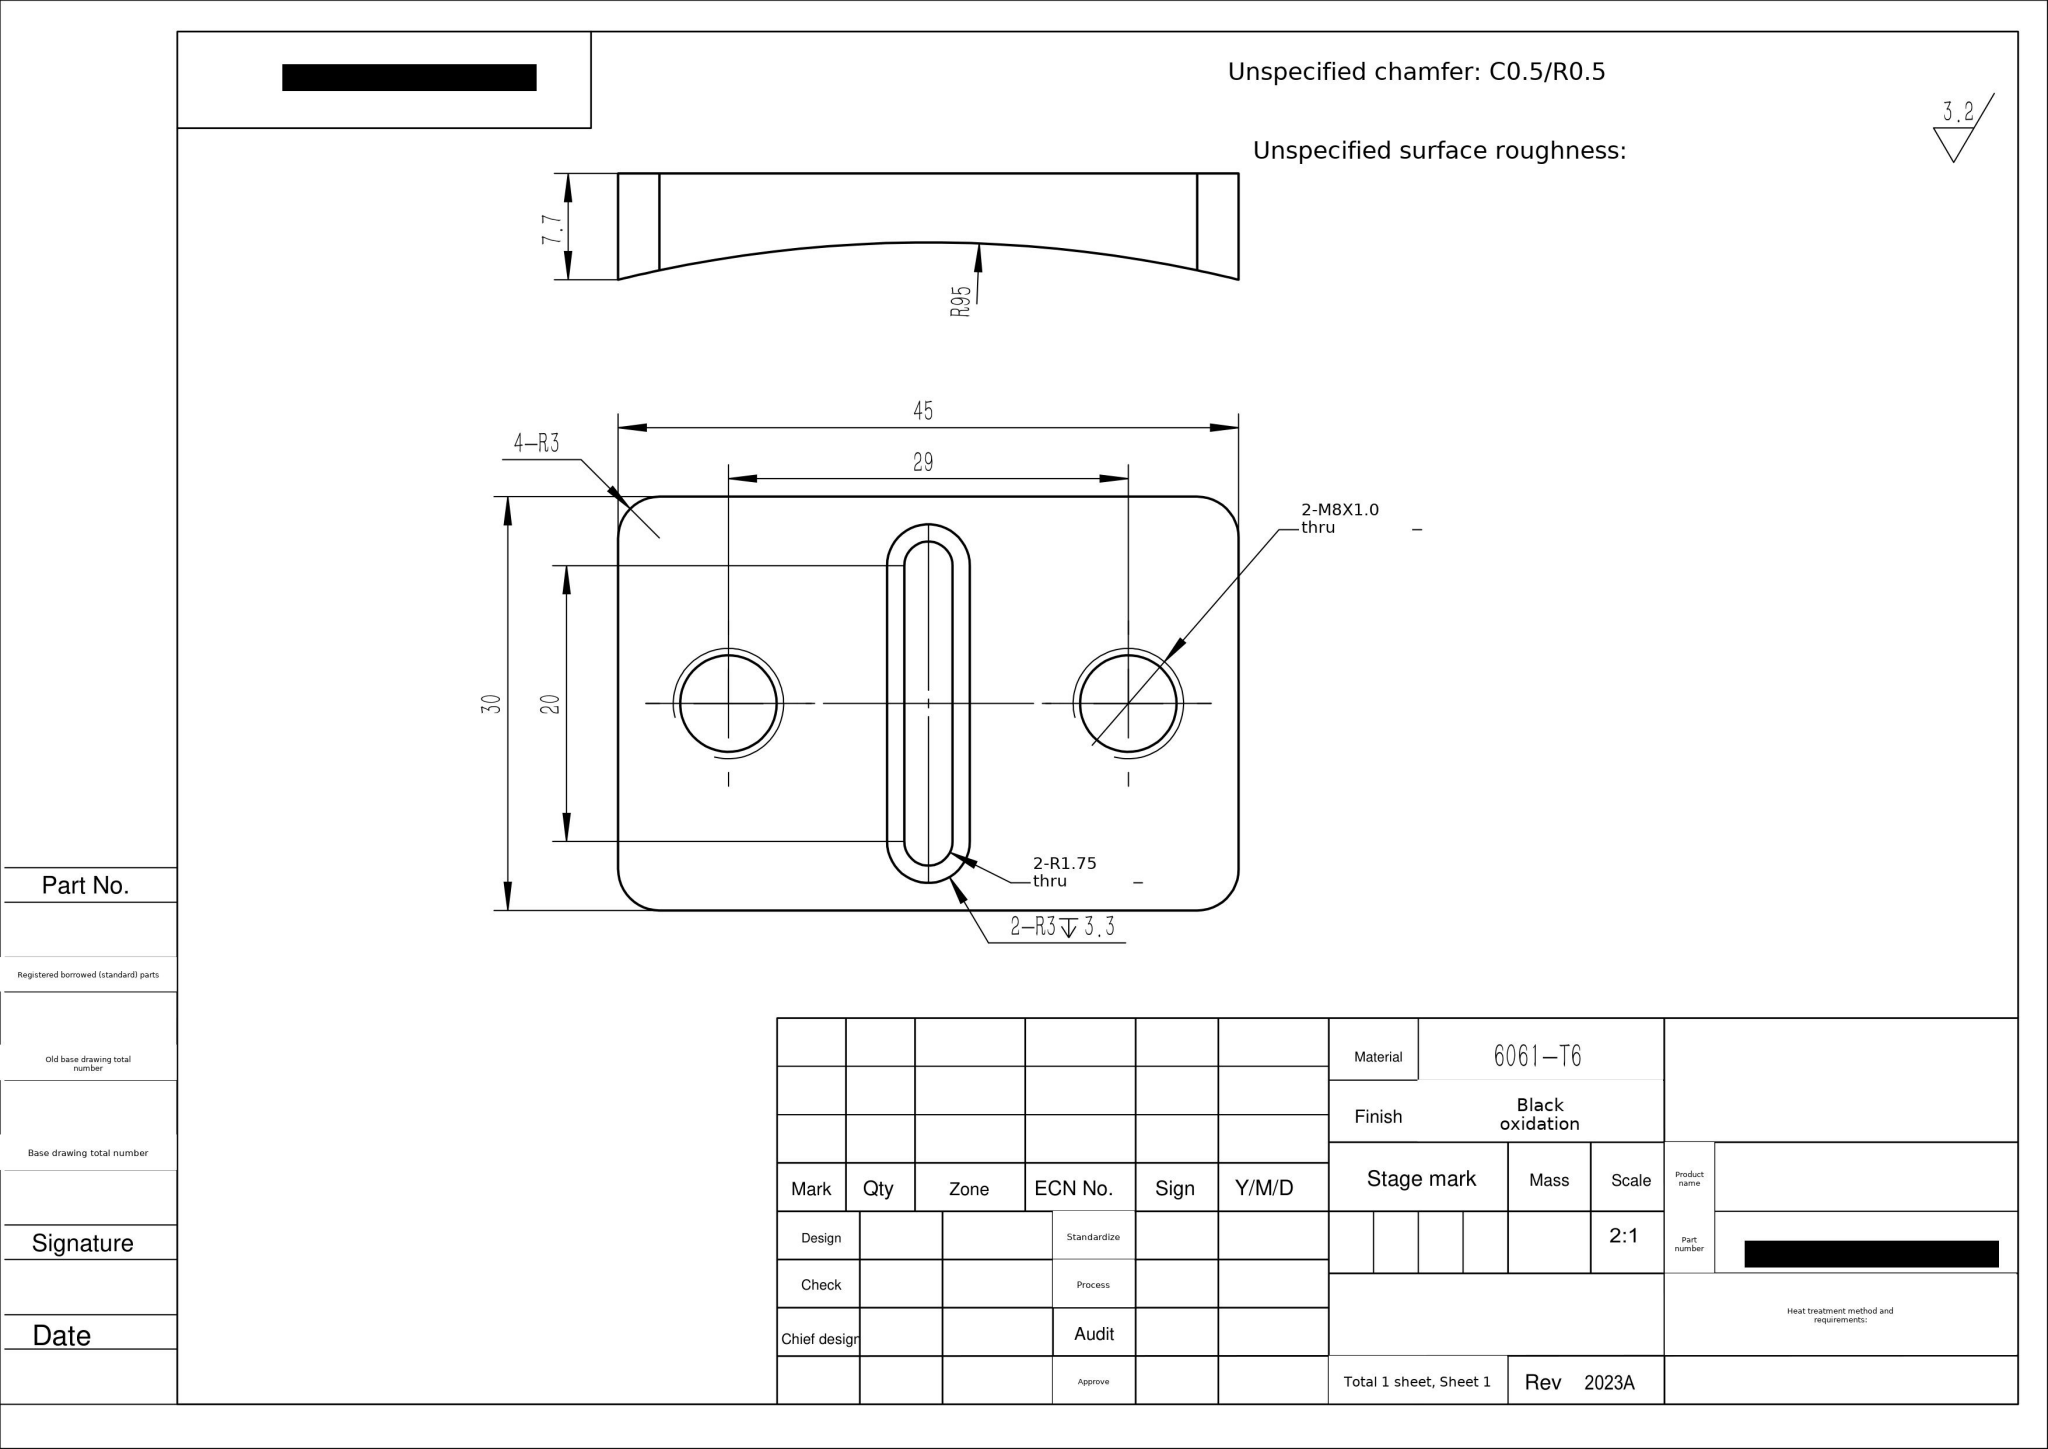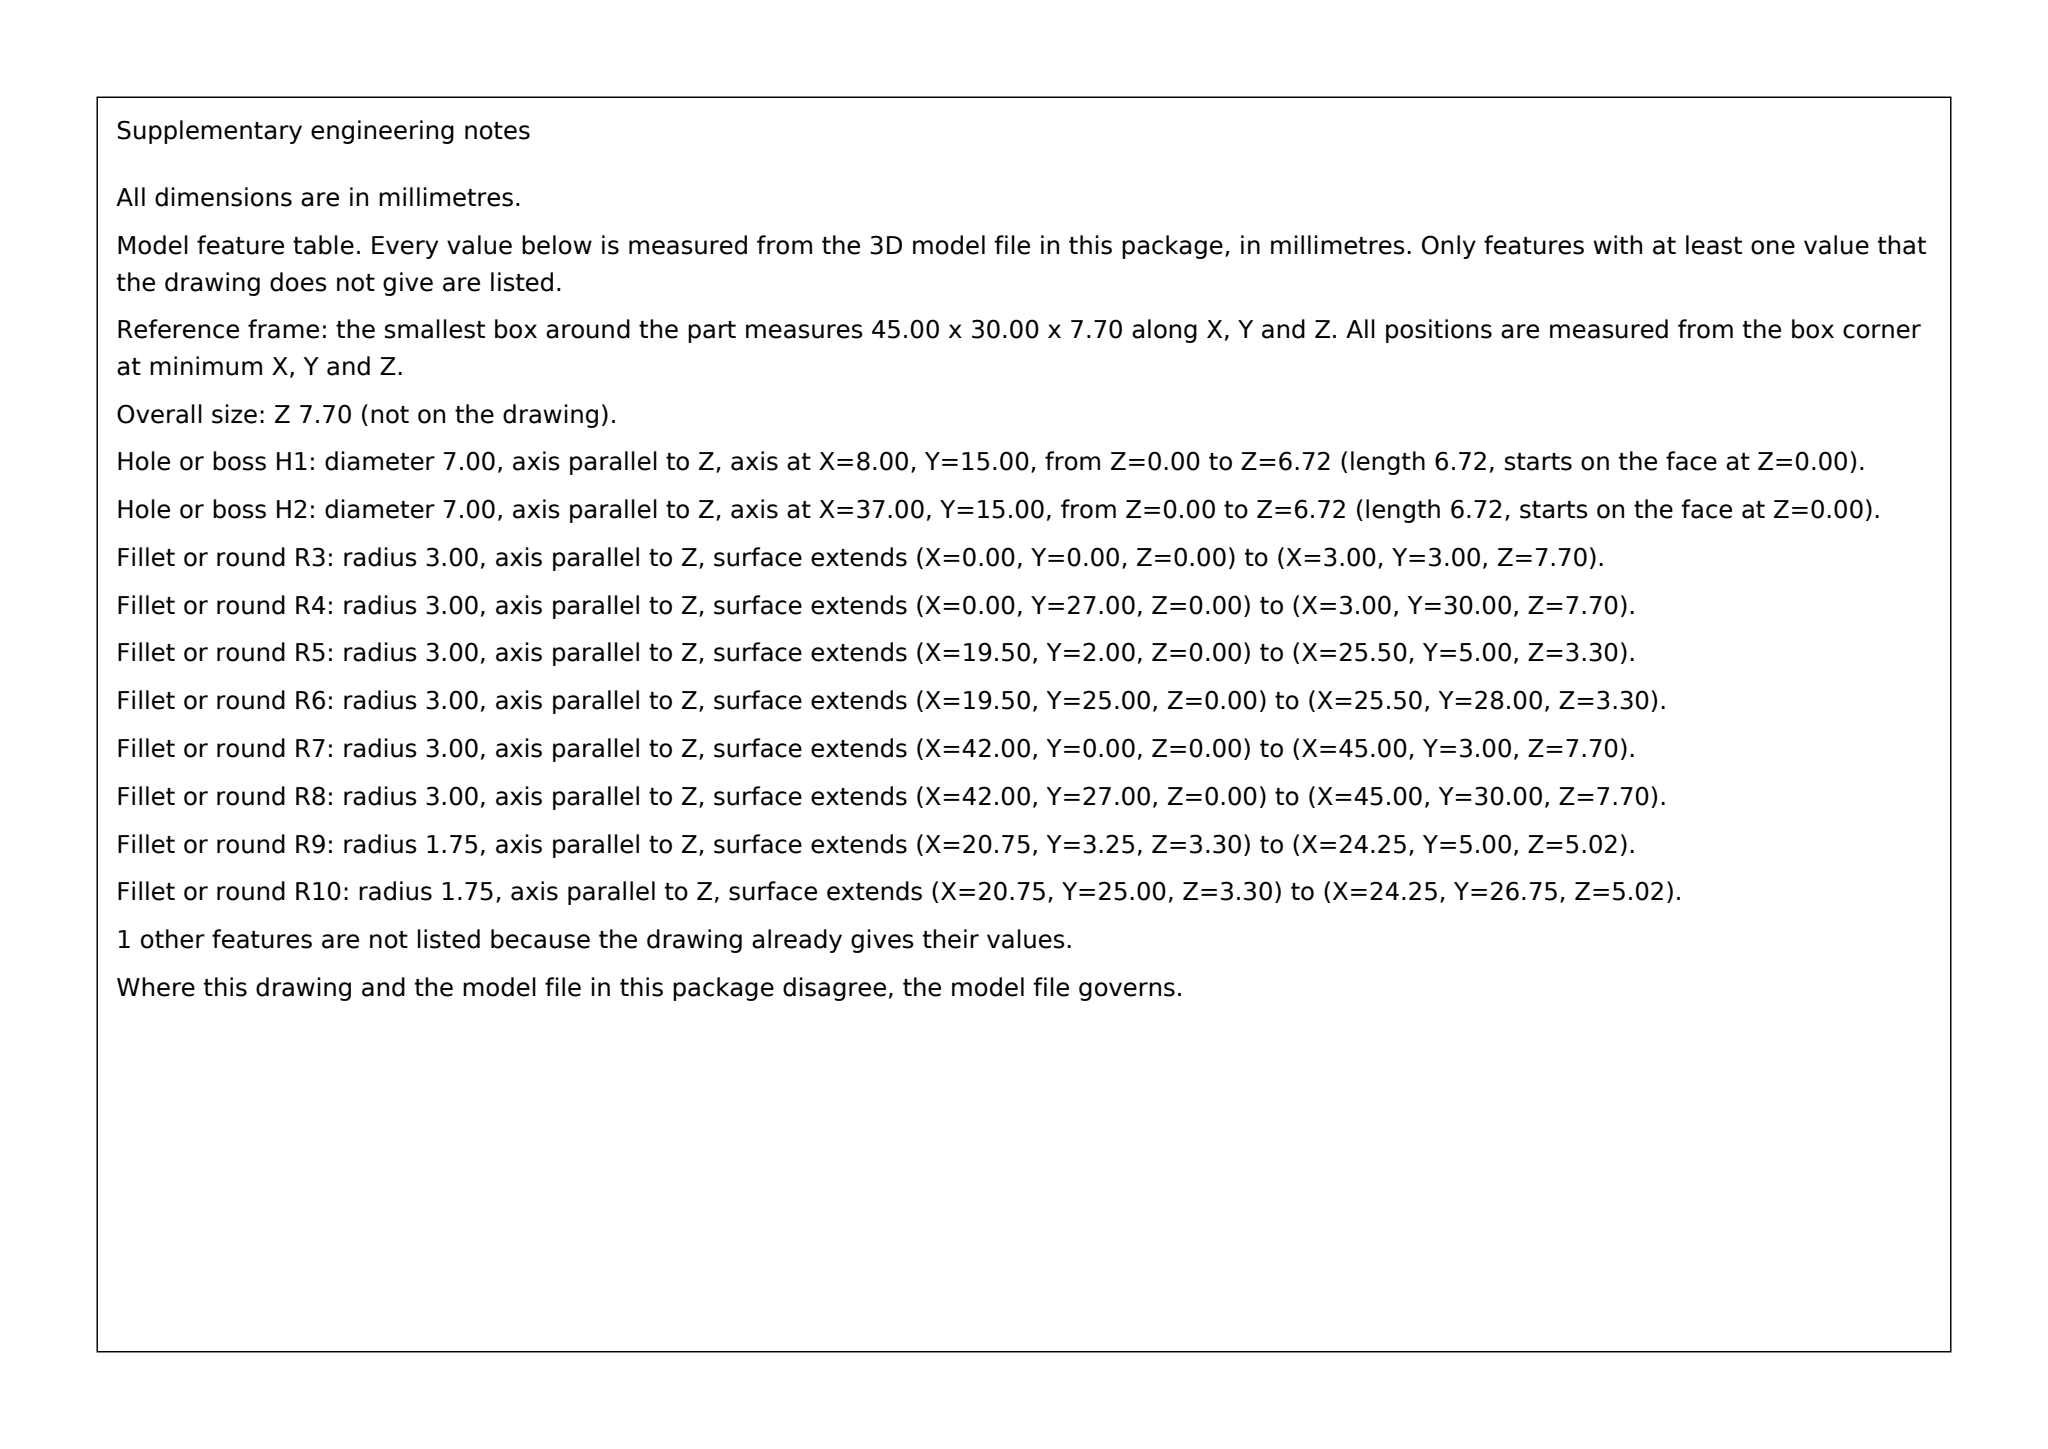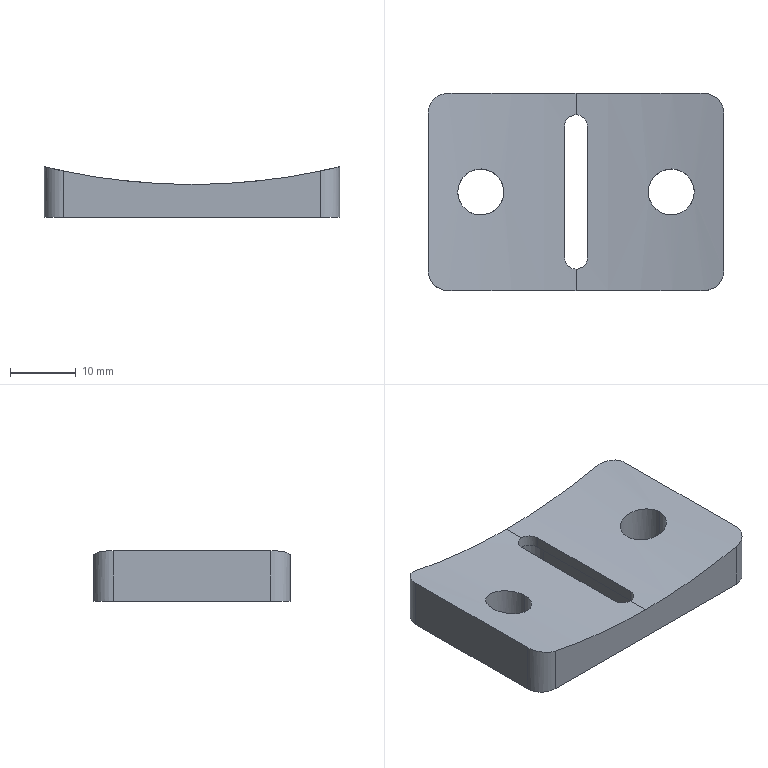Part | SolidWorks | mm | material 6061-T6 | 1 solid | 24 faces | box 45 x 30 x 7.7 mm | volume 6804 mm3 | cylinder 14 | plane 10 | commonest cylinder face diameters 6 x6 7 x4 190 x2 3.5 x2
build123d program:
from build123d import *

# Parameters (mm, degrees)
BOSS_EXTRUDE1_DEPTH   = 30
M8X1_0_TAPPED_HOLE1_D = 7
CUT_EXTRUDE1_DEPTH    = 39.283
CUT_EXTRUDE2_DEPTH    = 3.3
FILLET1_R             = 3


with BuildPart() as part:
    # Sketch1 → Boss-Extrude1 (new body)
    with BuildSketch(Plane(origin=(0, 0, 0), x_dir=(1, 0, 0), z_dir=(0, 1, 0))):
        with BuildLine():
            Line((-22.5, 92.297), (-22.5, 100))
            Line((-22.5, 100), (22.5, 100))
            Line((22.5, 100), (22.5, 92.297))
            ThreePointArc((22.5, 92.297), (0, 95), (-22.5, 92.297))
        make_face()
    extrude(amount=BOSS_EXTRUDE1_DEPTH)

    # M8x1.0 Tapped Hole1 (through all)
    with Locations(Plane(origin=(0, 0, -100), x_dir=(-1, 0, 0), z_dir=(0, 0, -1))):
        with Locations((-14.5, 15), (14.5, 15)):
            Hole(M8X1_0_TAPPED_HOLE1_D / 2)

    # Sketch4 → Cut-Extrude1 (cut, through all)
    with BuildSketch(Plane(origin=(0, 0, -100), x_dir=(-1, 0, 0), z_dir=(0, 0, -1))):
        with BuildLine():
            Line((1.75, 25), (1.75, 5))
            ThreePointArc((1.75, 5), (0, 3.25), (-1.75, 5))
            Line((-1.75, 5), (-1.75, 25))
            ThreePointArc((-1.75, 25), (0, 26.75), (1.75, 25))
        make_face()
    extrude(amount=-CUT_EXTRUDE1_DEPTH, mode=Mode.SUBTRACT)

    # Sketch5 → Cut-Extrude2 (cut)
    with BuildSketch(Plane(origin=(0, 0, -100), x_dir=(-1, 0, 0), z_dir=(0, 0, -1))):
        with BuildLine():
            Line((3, 25), (3, 5))
            ThreePointArc((3, 5), (0, 2), (-3, 5))
            Line((-3, 5), (-3, 25))
            ThreePointArc((-3, 25), (0, 28), (3, 25))
        make_face()
    extrude(amount=-CUT_EXTRUDE2_DEPTH, mode=Mode.SUBTRACT)

    # Fillet1
    fillet1_edges = [part.edges().sort_by_distance(p)[0] for p in [
        (22.5, 30, -96.149),
        (22.5, 0, -96.149),
        (-22.5, 0, -96.149),
        (-22.5, 30, -96.149),
    ]]
    fillet(fillet1_edges, radius=FILLET1_R)


solid = part.part